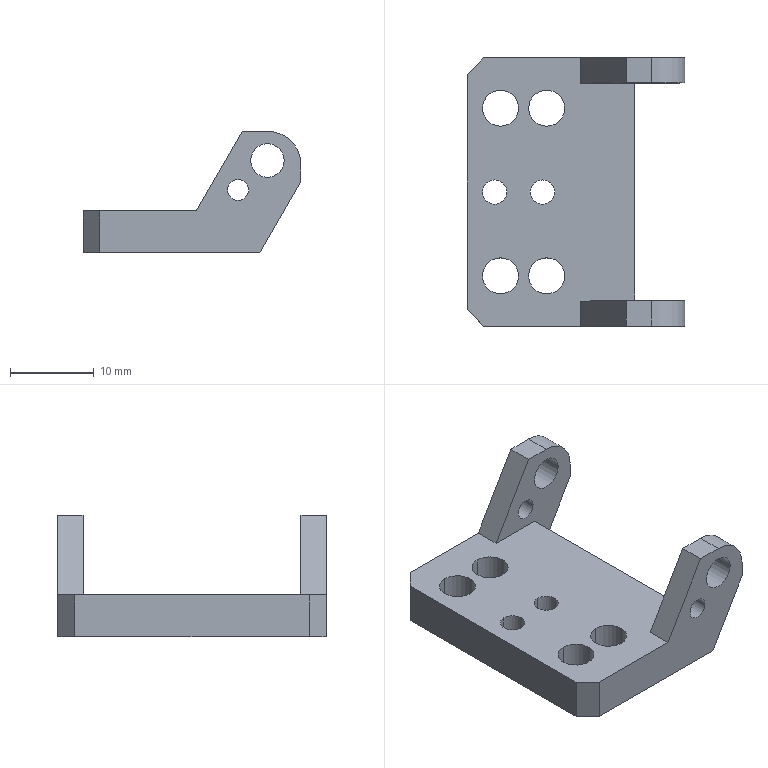Component | SolidWorks | 31298290203SupportFinger-1 | 1 solid | 46 faces | box 26 x 32 x 14.5 mm | volume 3205 mm3 | cylinder 26 | plane 20 | commonest cylinder face diameters 4.3 x8 2.5 x4 4 x4 5.5 x4 2.9 x4 8 x2 | material Q235-A
build123d program:
from build123d import *

# Parameters (mm, degrees)
BOSS_EXTRUDE1_DEPTH                               = 16
M2_5_HEX_SOCKET_HEAD_CAP_SCREW_CBORE1_D           = 2.9
M2_5_HEX_SOCKET_HEAD_CAP_SCREW_CBORE1_CBORE_D     = 5.5
M2_5_HEX_SOCKET_HEAD_CAP_SCREW_CBORE1_CBORE_DEPTH = 3
SKETCH4_R                                         = 2
CUT_EXTRUDE1_DEPTH                                = 44.706
FILLET1_R                                         = 4
SKETCH5_W                                         = 26
SKETCH5_H                                         = 9.5
CUT_EXTRUDE2_DEPTH                                = 34.797
CHAMFER1_SIZE                                     = 2
M3_TAPPED_HOLE1_D                                 = 2.5
SKETCH6_W                                         = 3.979
SKETCH6_H                                         = 26
CUT_EXTRUDE3_DEPTH                                = 34.797
F_4_3_4_3_DIAMETER_HOLE1_D                        = 4.3


with BuildPart() as part:
    # Sketch1 → Boss-Extrude1 (new, symmetric)
    with BuildSketch(Plane.XY):
        Polygon((0, 0), (21.093, 0), (26, -8.5), (26, -14.5), (19, -14.5), (13.515, -5), (0, -5), align=None)
    extrude(amount=BOSS_EXTRUDE1_DEPTH, both=True)

    # M2.5 Hex Socket Head Cap Screw CBORE1 (through all)
    with Locations(Plane(origin=(0, 0, 0), x_dir=(-1, 0, 0), z_dir=(0, 1, 0))):
        with Locations((-3.3, 0), (-9, 0)):
            CounterBoreHole(M2_5_HEX_SOCKET_HEAD_CAP_SCREW_CBORE1_D / 2, M2_5_HEX_SOCKET_HEAD_CAP_SCREW_CBORE1_CBORE_D / 2, M2_5_HEX_SOCKET_HEAD_CAP_SCREW_CBORE1_CBORE_DEPTH)

    # Sketch4 → Cut-Extrude1 (cut, through all)
    with BuildSketch(Plane(origin=(0, 0, -16), x_dir=(-1, 0, 0), z_dir=(0, 0, -1))):
        with Locations((-22, -11)):
            Circle(SKETCH4_R)
    extrude(amount=-CUT_EXTRUDE1_DEPTH, mode=Mode.SUBTRACT)

    # Fillet1
    fillet1_edges = [part.edges().sort_by_distance(p)[0] for p in [
        (26, -14.5, 0),
    ]]
    fillet(fillet1_edges, radius=FILLET1_R)

    # Sketch5 → Cut-Extrude2 (cut, through all)
    with BuildSketch(Plane(origin=(26, 0, 0), x_dir=(0, 0, -1), z_dir=(1, 0, 0))):
        with Locations((0, -9.75)):
            Rectangle(SKETCH5_W, SKETCH5_H)
    extrude(amount=-CUT_EXTRUDE2_DEPTH, mode=Mode.SUBTRACT)

    # Chamfer1
    chamfer1_edges = [part.edges().sort_by_distance(p)[0] for p in [
        (0, -2.5, 16),
        (0, -2.5, -16),
    ]]
    chamfer(chamfer1_edges, length=CHAMFER1_SIZE)

    # M3 Tapped Hole1 (through all)
    with Locations(Plane(origin=(0, 0, -16), x_dir=(-1, 0, 0), z_dir=(0, 0, -1))):
        with Locations((-18.5, -7.5)):
            Hole(M3_TAPPED_HOLE1_D / 2)

    # Sketch6 → Cut-Extrude3 (cut, through all)
    with BuildSketch(Plane(origin=(0, 0, 0), x_dir=(1, 0, 0), z_dir=(0, 1, 0))):
        with Locations((21.99, 0)):
            Rectangle(SKETCH6_W, SKETCH6_H)
    extrude(amount=-CUT_EXTRUDE3_DEPTH, mode=Mode.SUBTRACT)

    # 4.3 _4.3_ Diameter Hole1 (through all)
    with Locations(Plane(origin=(0, 0, 0), x_dir=(-1, 0, 0), z_dir=(0, 1, 0))):
        with Locations((-4, -10), (-9.5, -10), (-4, 10), (-9.5, 10)):
            Hole(F_4_3_4_3_DIAMETER_HOLE1_D / 2)


solid = part.part

# Placed as in the assembly
solid = solid.moved(Location((188.87, 43.668, 23.729), (-90, 0, 0)))